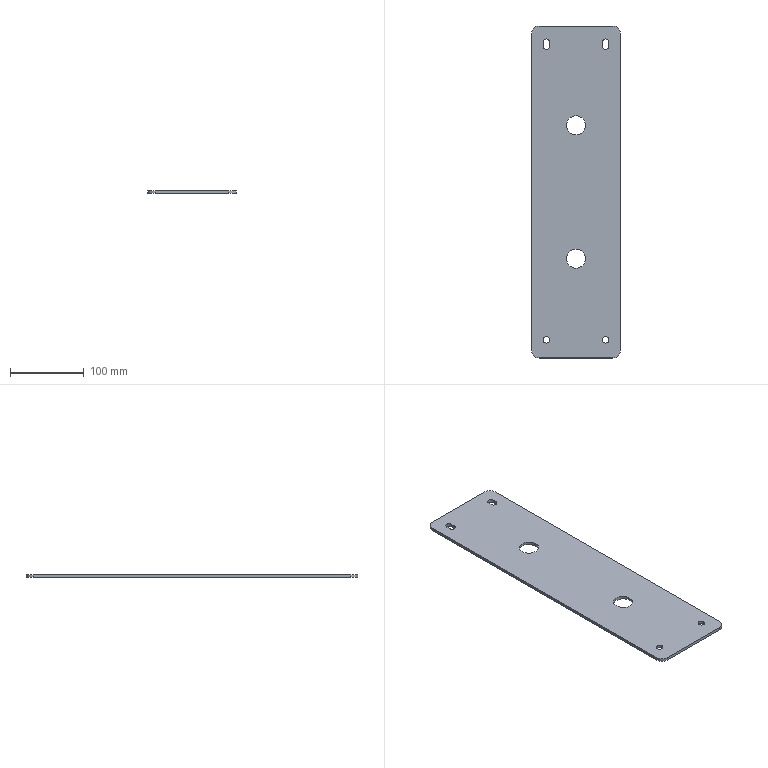CAM job | Mastercam | mm | 1 operations | part box 120 x 449 x 4
1. Contour (2D chamfer) | 7 - 12 倒角刀